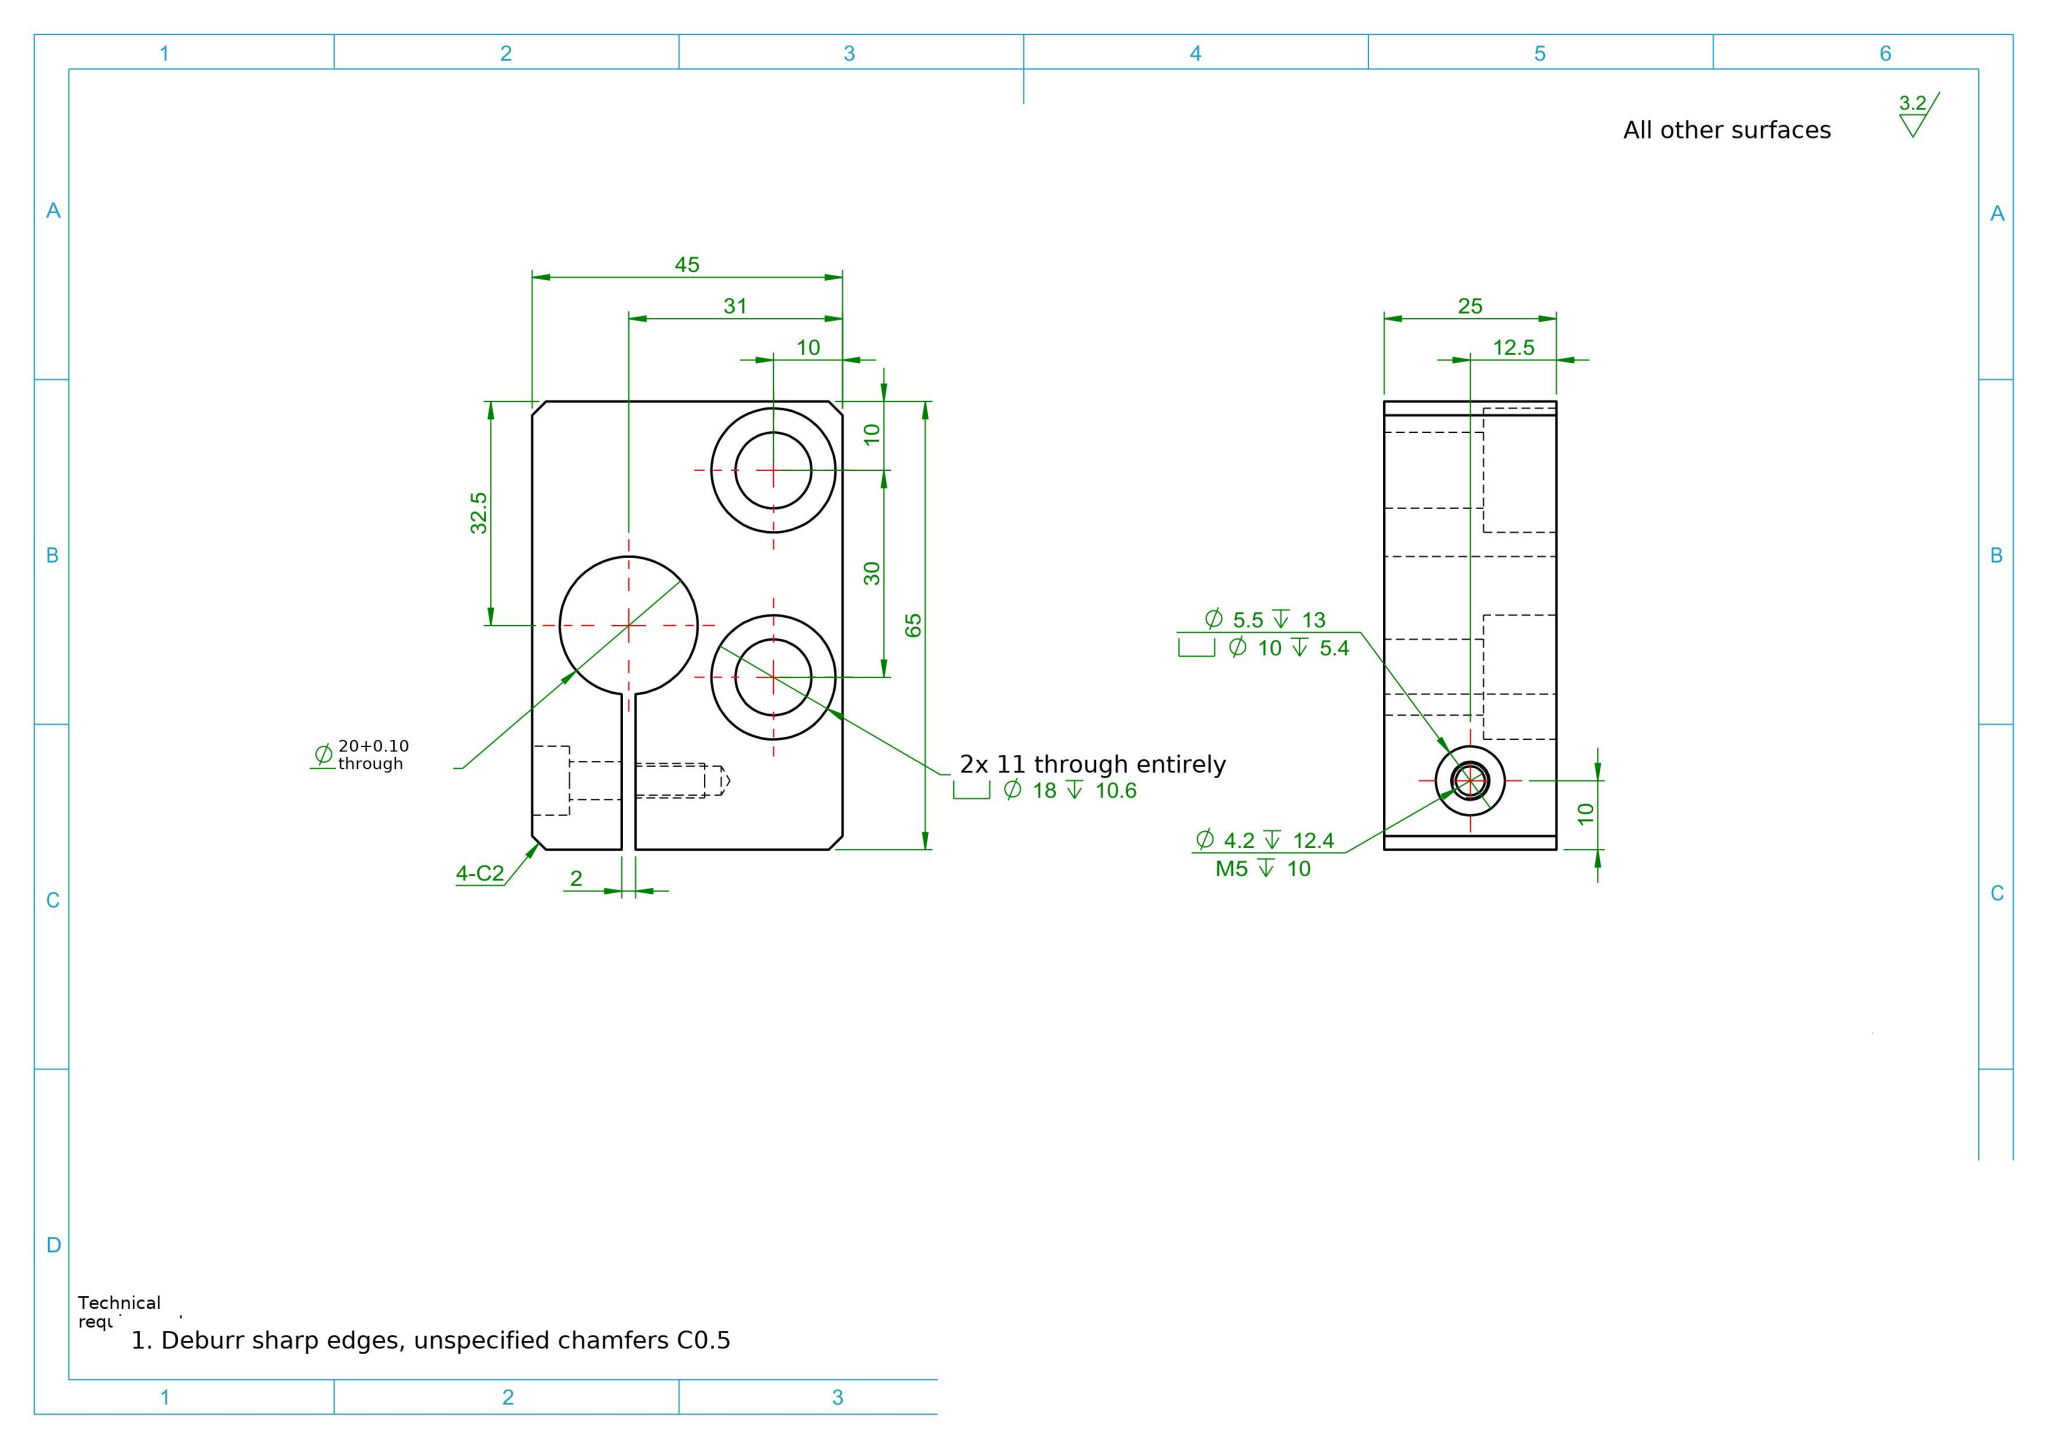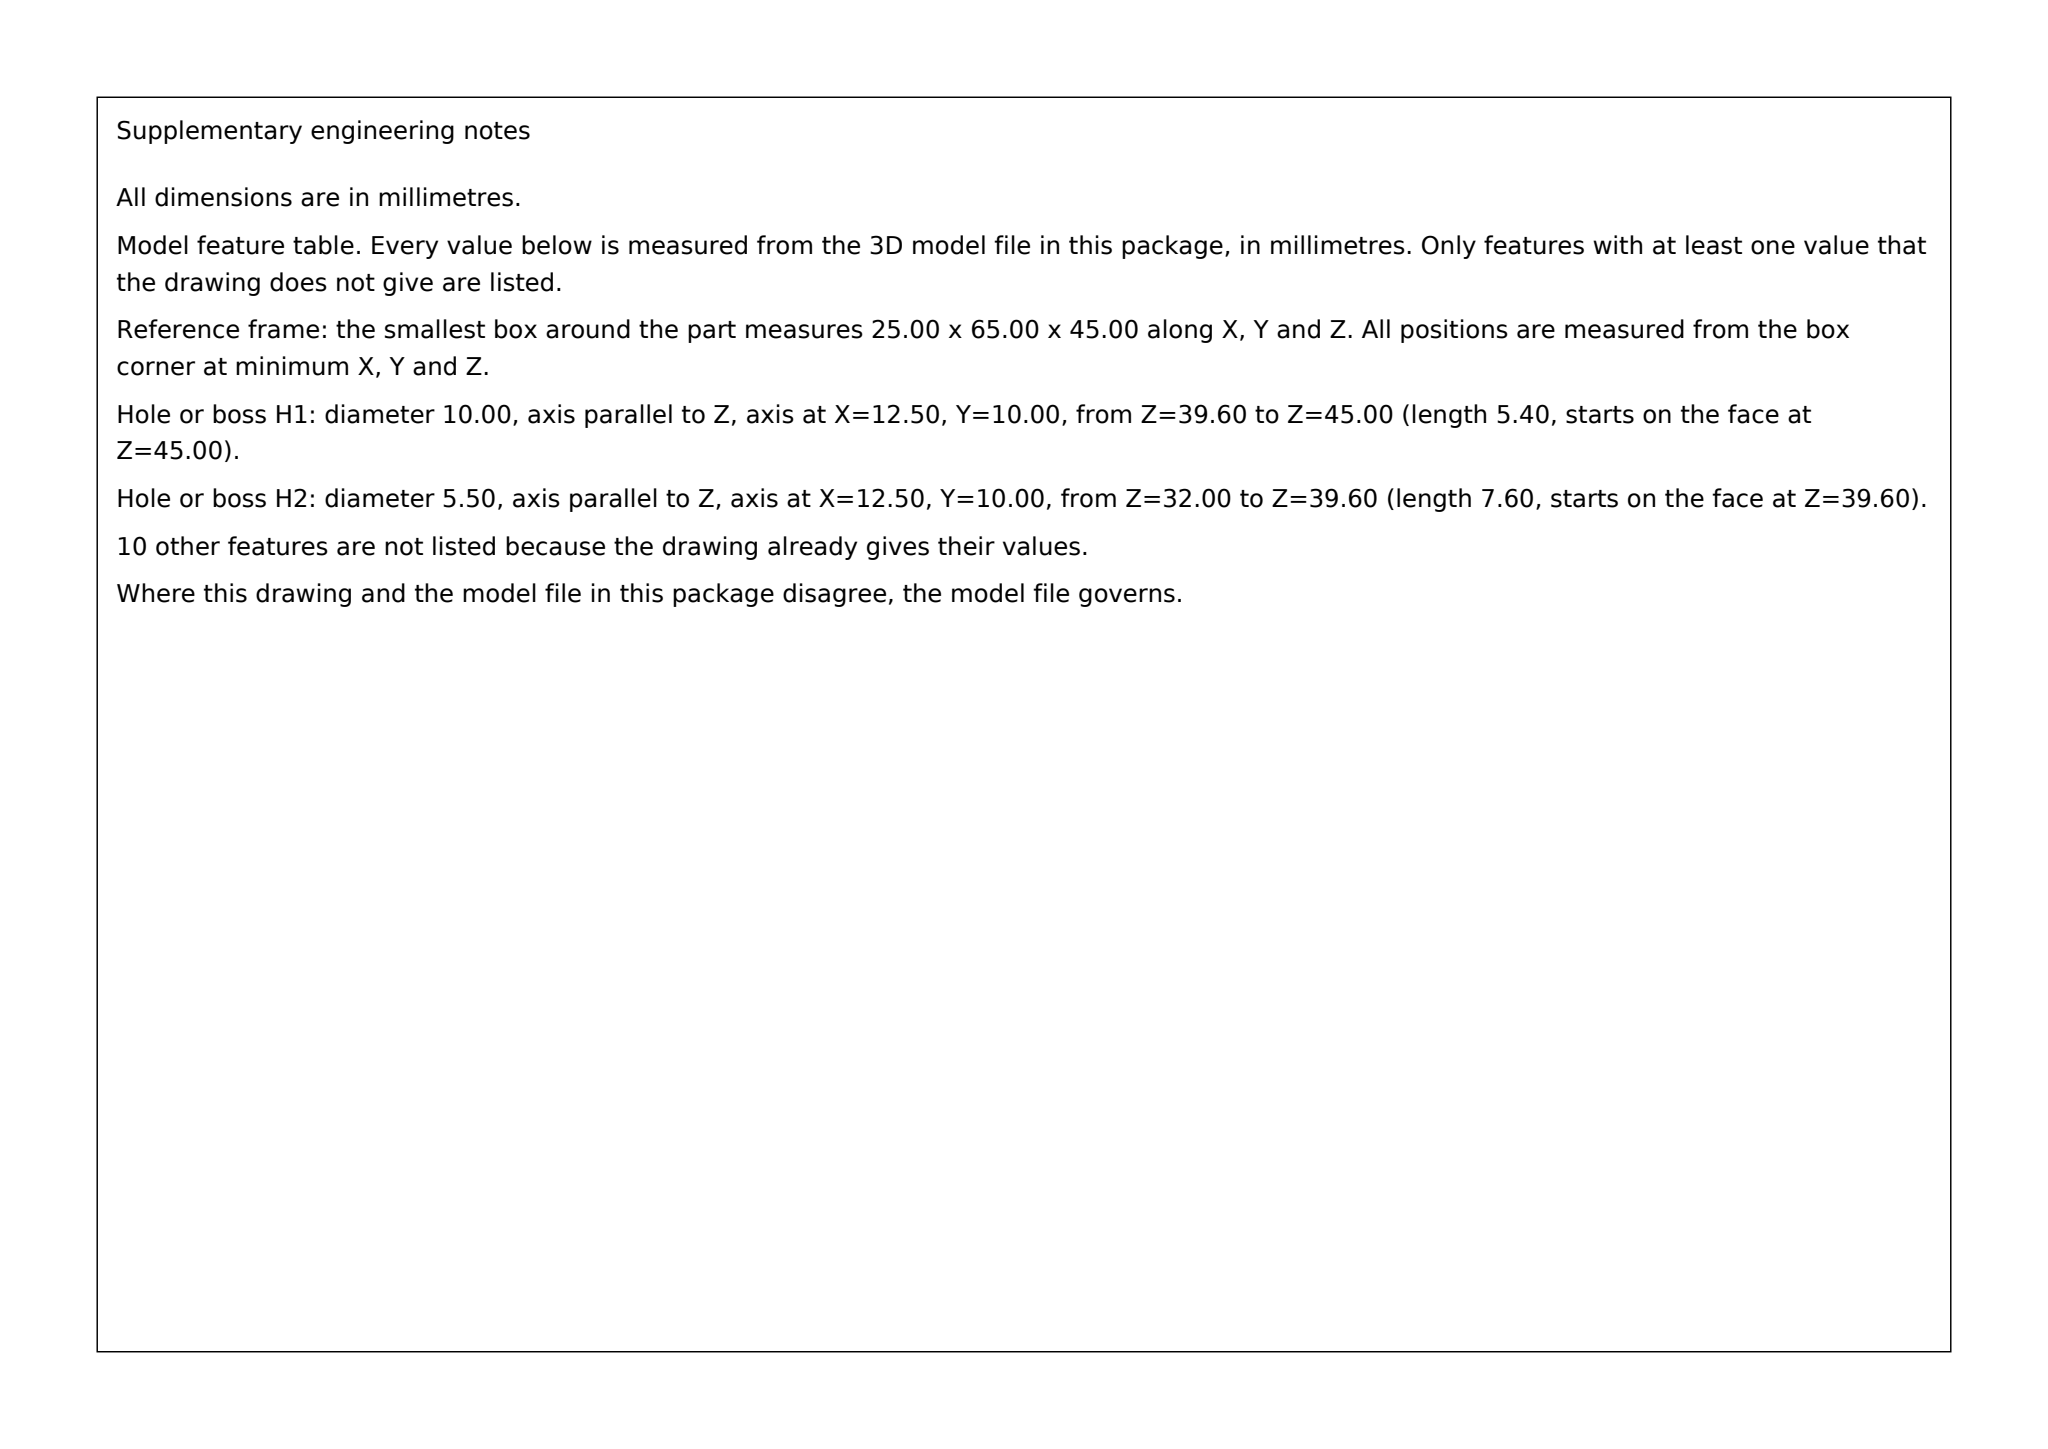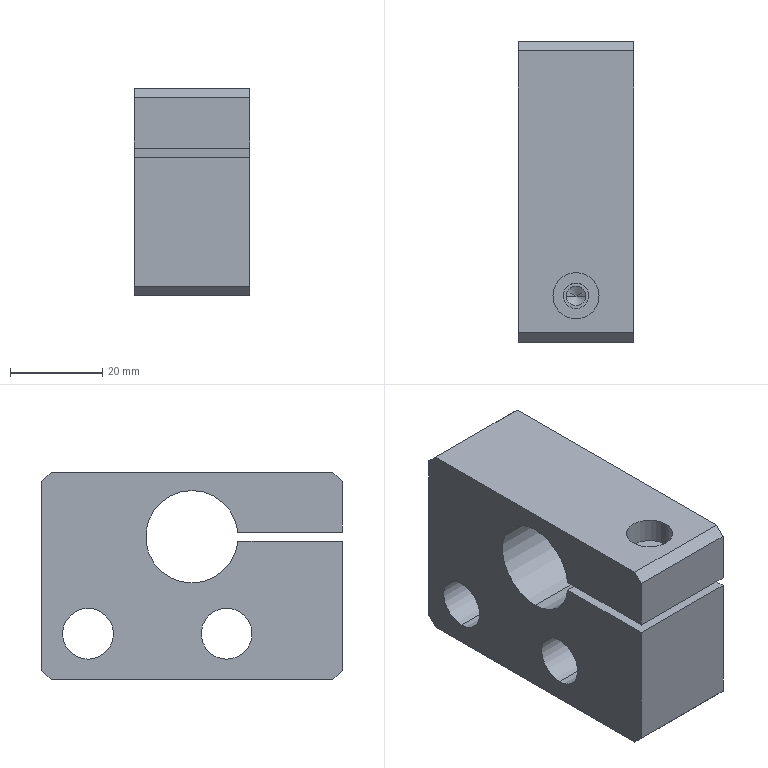Part | SolidWorks | mm | 1 solid | 35 faces | box 25 x 65 x 45 mm | volume 55031 mm3 | cylinder 17 | plane 16 | cone 2 | commonest cylinder face diameters 18 x4 11 x4 20 x3 4.2 x2 10 x2 5.5 x2